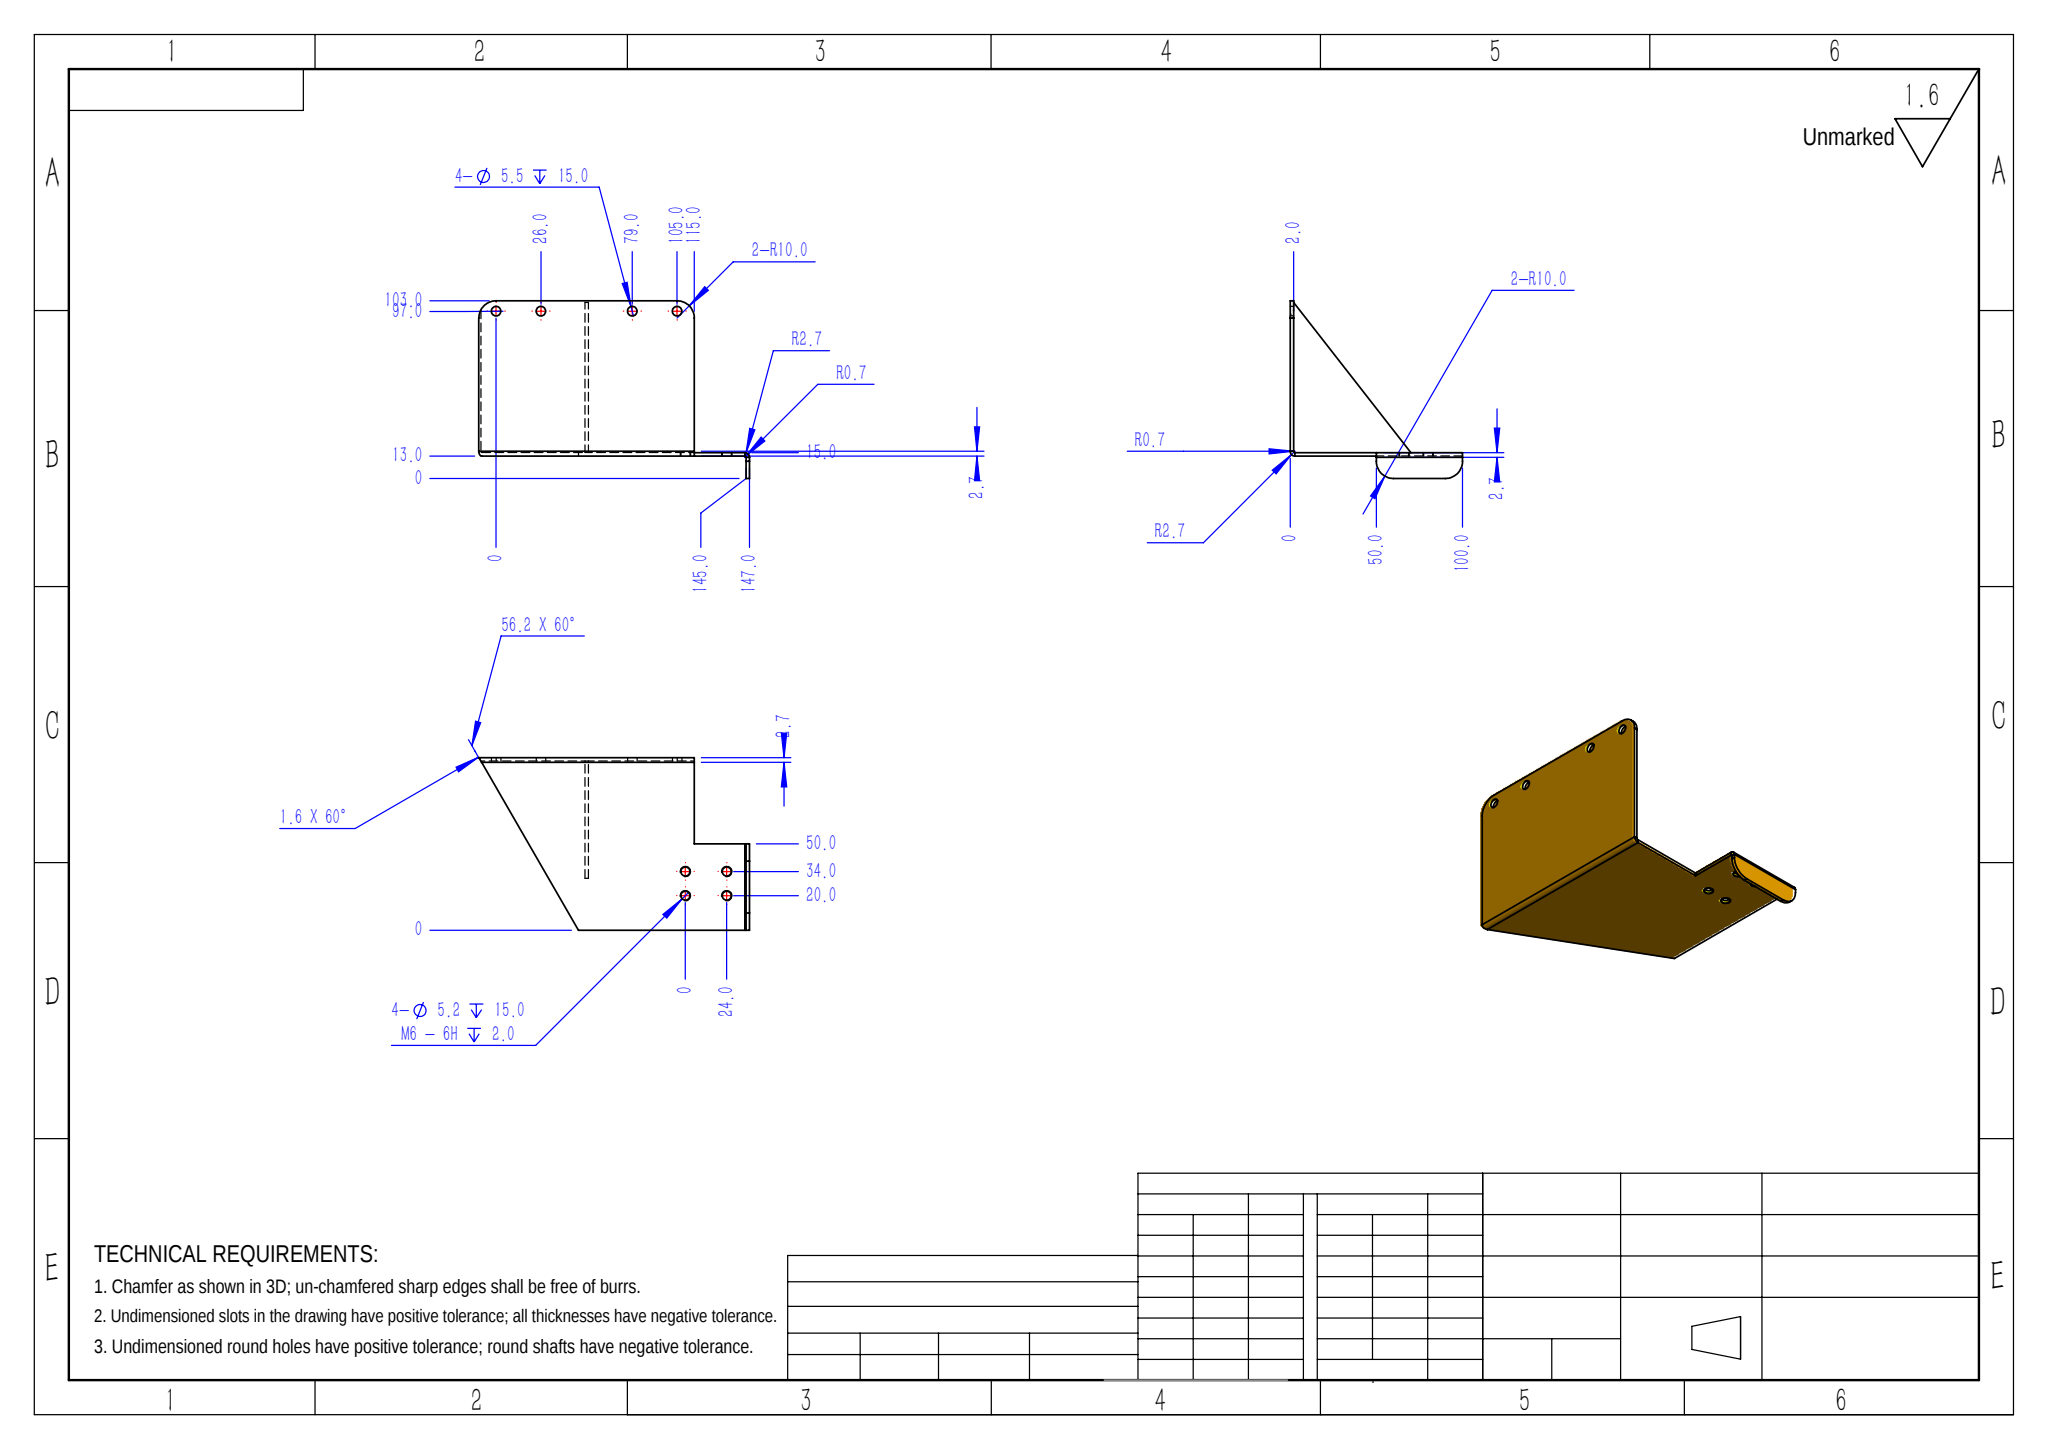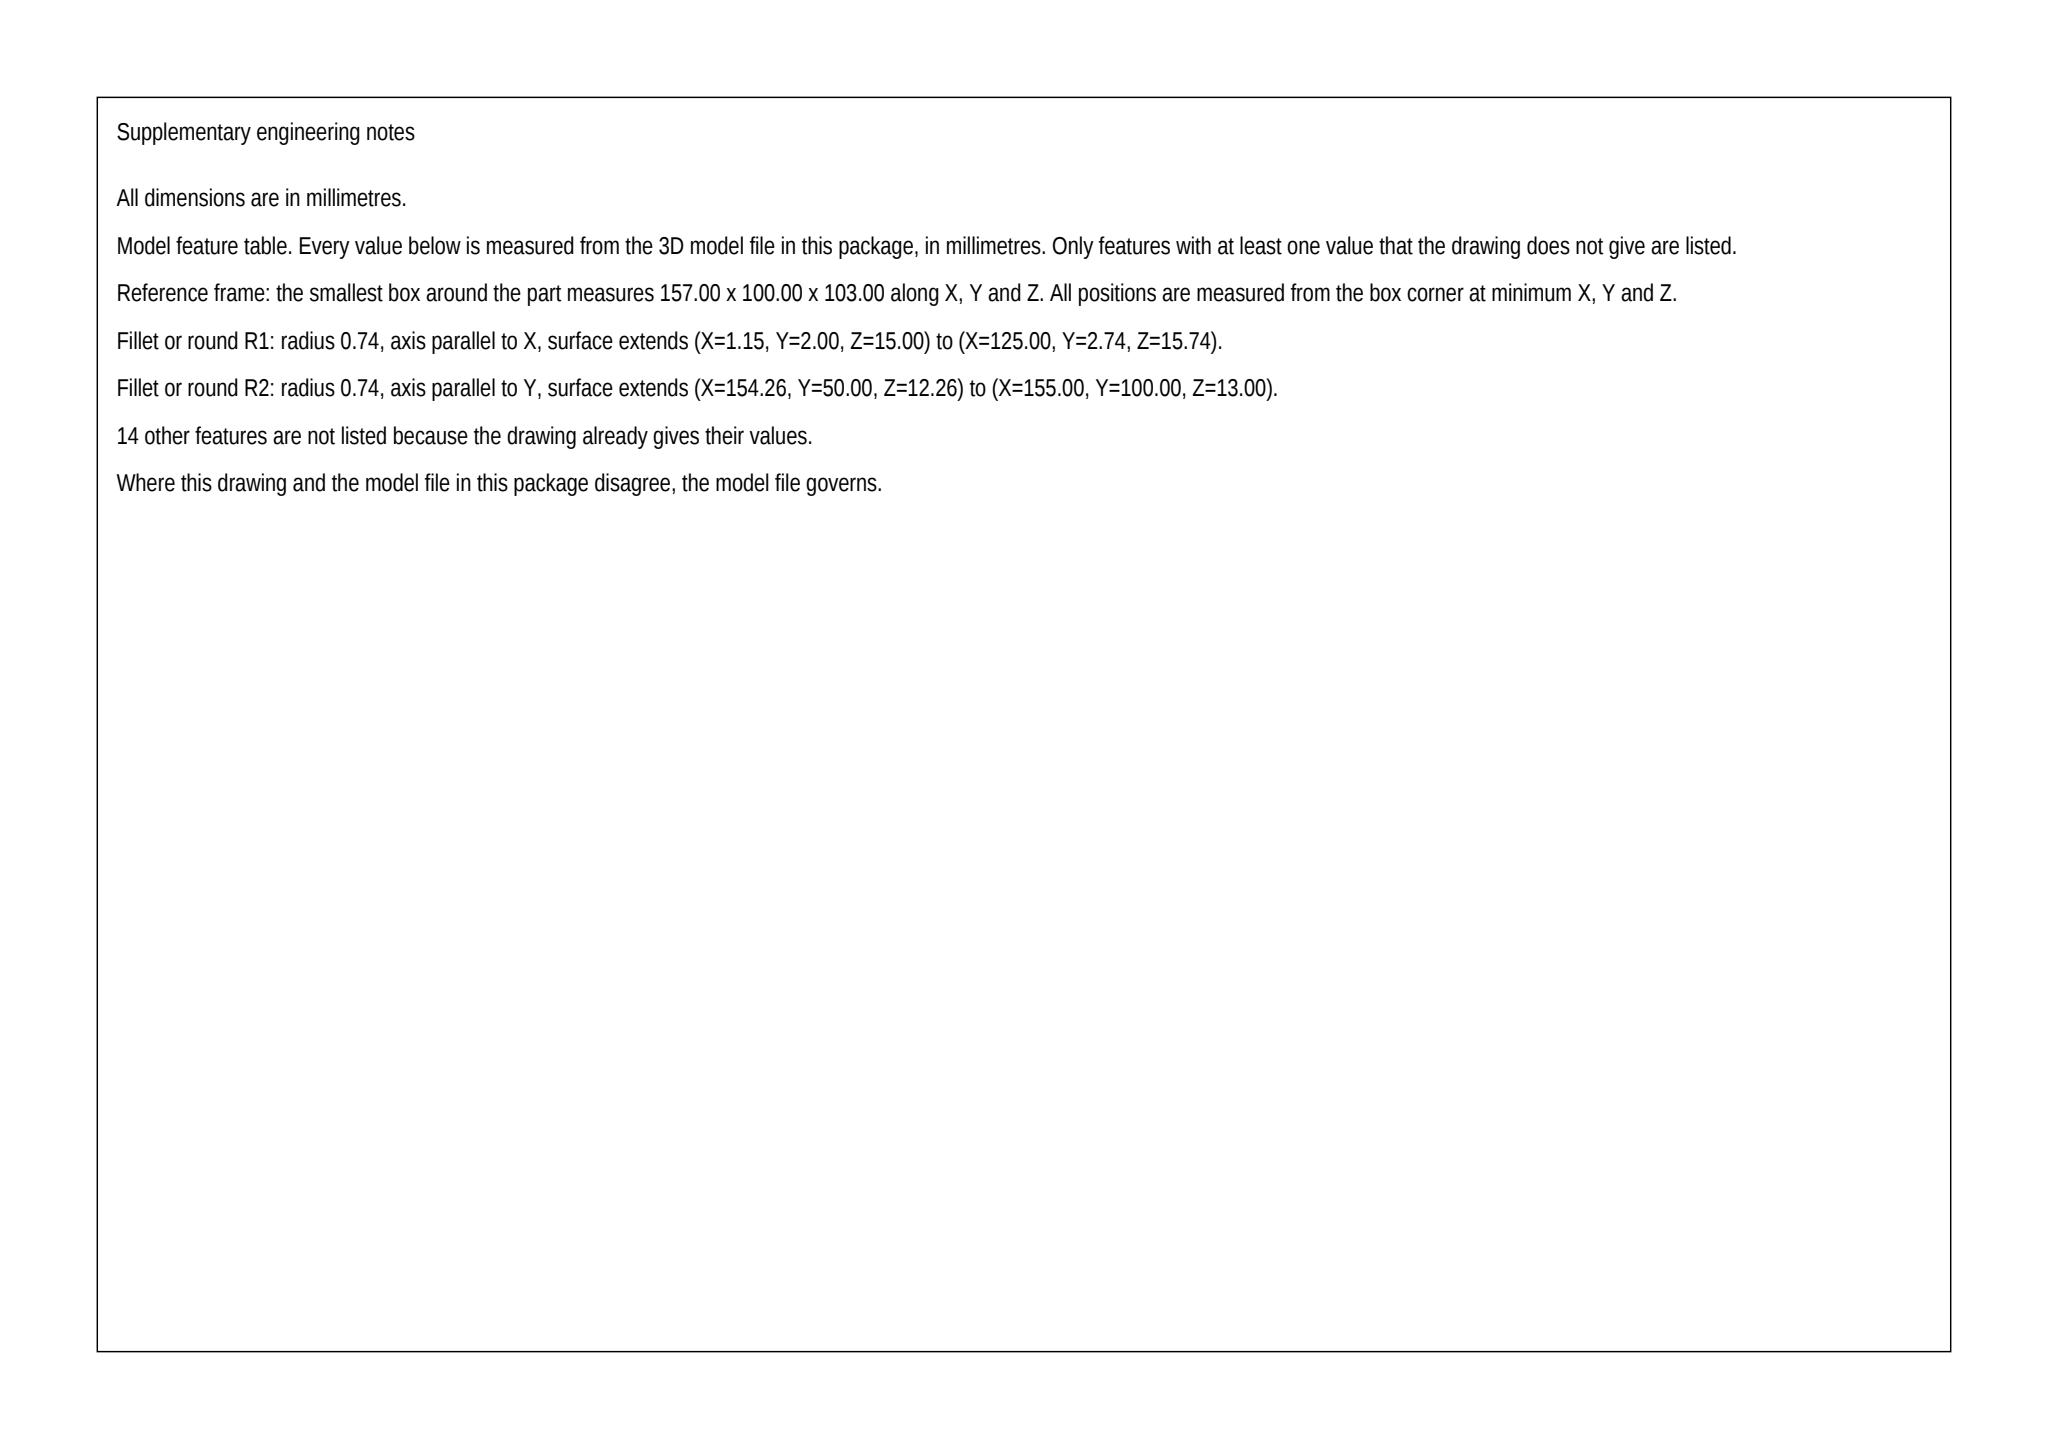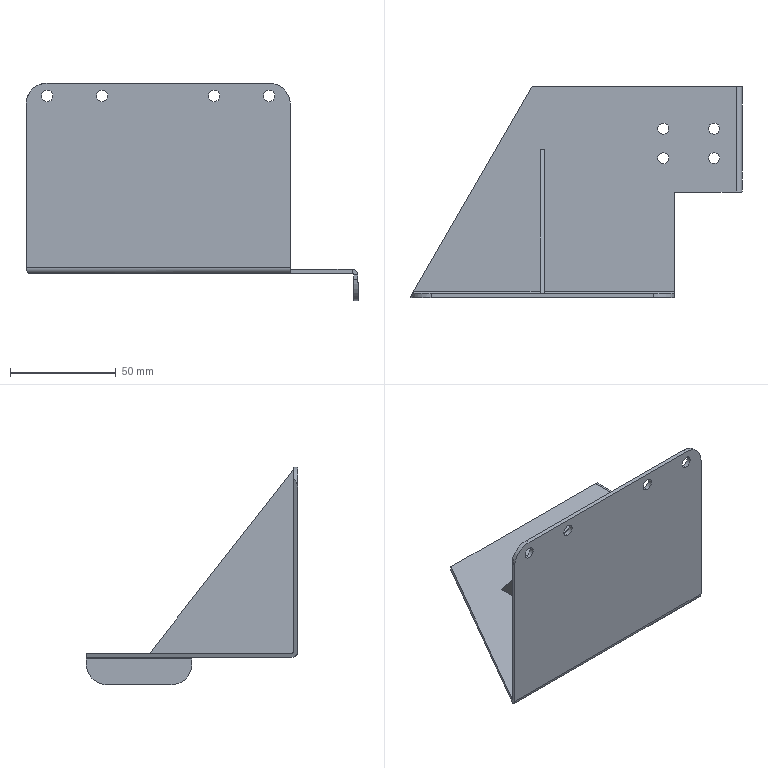Part | SolidWorks | mm | 1 solid | 46 faces | box 157 x 100 x 103 mm | volume 50757 mm3 | cylinder 25 | plane 21 | commonest cylinder face diameters 5.5 x8 5.2 x8 20 x4 1.473 x3 5.473 x2
Drawing notes:
OVERALL 157.0 X 100.0 X 103.0 | from the solid: bbox_xyz [157.0, 100.0, 103.0]
MATL THK 2.0 TYP; BEND R0.7 INSIDE / R2.7 OUTSIDE | from the solid: y-planes 0.0 & 2.0 give 2.0 wall; bend cyls Ø1.473 (R0.74) inner, Ø5.473 (R2.74) outer
FRONT VIEW: 4-Ø5.5 HOLE ROW CL 97.0 ABV 0 DATUM (BTM EDGE) | from the solid: Ø5.5 y-axis holes at x=10/36/89/115, z=96.98; bbox z-min=0 is the 0 datum
2-R10.0 AT FLANGE BTM CORNERS, CL 60.0 & 90.0, 10.0 ABV 0 | from the solid: Ø20 x-axis cyls at y=60 & y=90, z=10, length 2.0 (flange thk)
4-Ø5.2/M6 PATTERN X: 109.8 & 133.8 FROM 0 DATUM OF TOP VIEW | from the solid: Ø5.2 holes at x=119.8 & 143.8; top-view 0 datum = 1st Ø5.5 hole at x=10.0 (right edge x=157 shown as 147.0)